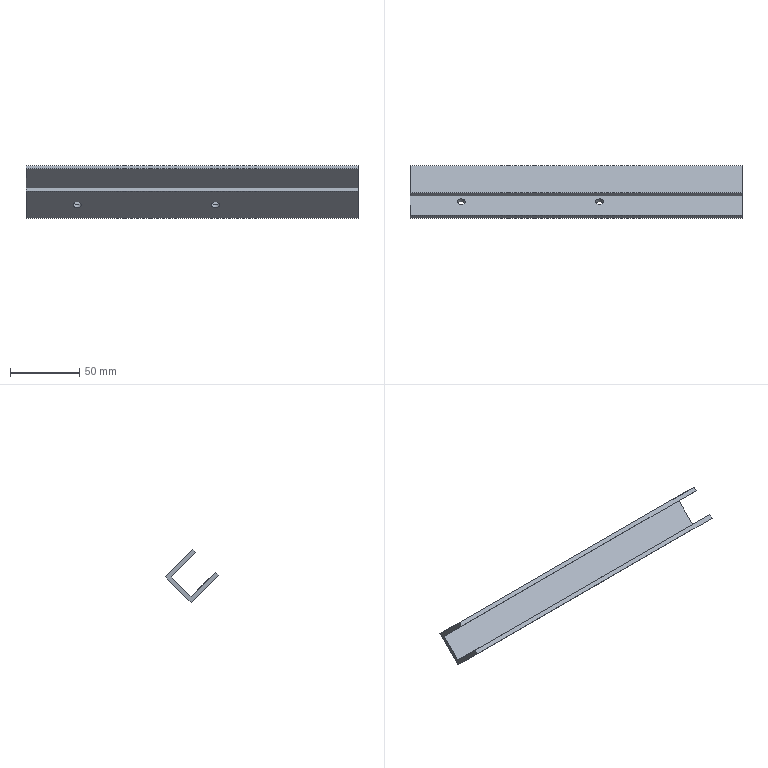Component | SolidWorks | Bracket-1 | 1 solid | 14 faces | box 240 x 38.18 x 38.18 mm | volume 54550 mm3 | plane 10 | cylinder 4 | commonest cylinder face diameters 6 x4
build123d program:
from build123d import *

# Parameters (mm, degrees)
EXTRUDE_THIN1_DEPTH = 240
SKETCH3_R           = 3
CUT_EXTRUDE1_DEPTH  = 3


with BuildPart() as part:
    # Sketch1 → Extrude-Thin1 (new body)
    with BuildSketch(Plane.XY):
        Polygon((-53.556, 14.33), (-25.556, 14.33), (-25.556, -11.67), (-53.556, -11.67), (-53.556, -8.67), (-28.556, -8.67), (-28.556, 11.33), (-53.556, 11.33), align=None)
    extrude(amount=EXTRUDE_THIN1_DEPTH)

    # Sketch3 → Cut-Extrude1 (cut)
    with BuildSketch(Plane(origin=(0, 14.33, 0), x_dir=(1, 0, 0), z_dir=(0, 1, 0))):
        with Locations(Location((-39.556, -103, 0), (0, 0, 270))):
            Circle(SKETCH3_R)
        with Locations(Location((-39.556, -203, 0), (0, 0, 270))):
            Circle(SKETCH3_R)
    extrude(amount=-CUT_EXTRUDE1_DEPTH, mode=Mode.SUBTRACT)


solid = part.part

# Placed as in the assembly
solid = solid.moved(Location((728.45, -151.935, -266.823), (-135, -90, 0)))
STEP:
#1=COLOUR_RGB('',0.7922,0.8196,0.9333);
#2=FILL_AREA_STYLE_COLOUR('',#1);
#3=FILL_AREA_STYLE('',(#2));
#4=SURFACE_STYLE_FILL_AREA(#3);
#5=SURFACE_SIDE_STYLE('',(#4));
#6=SURFACE_STYLE_USAGE(.BOTH.,#5);
#7=PRESENTATION_STYLE_ASSIGNMENT((#6));
#8=CARTESIAN_POINT('',(20.805,-7.398,-9.719));
#9=VERTEX_POINT('',#8);
#10=CARTESIAN_POINT('',(20.569,-7.398,-9.719));
#11=VERTEX_POINT('',#10);
#12=CARTESIAN_POINT('',(20.687,-7.398,-9.719));
#13=DIRECTION('',(0.,-0.7071,-0.7071));
#14=DIRECTION('',(-1.,0.,0.));
#15=AXIS2_PLACEMENT_3D('',#12,#13,#14);
#16=CIRCLE('',#15,0.1181);
#17=EDGE_CURVE('',#9,#11,#16,.T.);
#18=ORIENTED_EDGE('',*,*,#17,.F.);
#19=CARTESIAN_POINT('',(20.805,-7.482,-9.803));
#20=VERTEX_POINT('',#19);
#21=CARTESIAN_POINT('',(20.805,-7.398,-9.719));
#22=DIRECTION('',(0.,-0.7071,-0.7071));
#23=VECTOR('',#22,39.37);
#24=LINE('',#21,#23);
#25=EDGE_CURVE('',#9,#20,#24,.T.);
#26=ORIENTED_EDGE('',*,*,#25,.T.);
#27=CARTESIAN_POINT('',(20.569,-7.482,-9.803));
#28=VERTEX_POINT('',#27);
#29=CARTESIAN_POINT('',(20.687,-7.482,-9.803));
#30=DIRECTION('',(0.,-0.7071,-0.7071));
#31=DIRECTION('',(-1.,0.,0.));
#32=AXIS2_PLACEMENT_3D('',#29,#30,#31);
#33=CIRCLE('',#32,0.1181);
#34=EDGE_CURVE('',#20,#28,#33,.T.);
#35=ORIENTED_EDGE('',*,*,#34,.T.);
#36=CARTESIAN_POINT('',(20.569,-7.398,-9.719));
#37=DIRECTION('',(0.,-0.7071,-0.7071));
#38=VECTOR('',#37,39.37);
#39=LINE('',#36,#38);
#40=EDGE_CURVE('',#11,#28,#39,.T.);
#41=ORIENTED_EDGE('',*,*,#40,.F.);
#42=EDGE_LOOP('',(#18,#26,#35,#41));
#43=FACE_OUTER_BOUND('',#42,.T.);
#44=CARTESIAN_POINT('',(20.687,-7.398,-9.719));
#45=DIRECTION('',(0.,-0.7071,-0.7071));
#46=DIRECTION('',(-1.,0.,0.));
#47=AXIS2_PLACEMENT_3D('',#44,#45,#46);
#48=CYLINDRICAL_SURFACE('',#47,0.1181);
#49=ADVANCED_FACE('',(#43),#48,.F.);
#50=CARTESIAN_POINT('',(24.742,-7.398,-9.719));
#51=VERTEX_POINT('',#50);
#52=CARTESIAN_POINT('',(24.506,-7.398,-9.719));
#53=VERTEX_POINT('',#52);
#54=CARTESIAN_POINT('',(24.624,-7.398,-9.719));
#55=DIRECTION('',(0.,-0.7071,-0.7071));
#56=DIRECTION('',(-1.,0.,0.));
#57=AXIS2_PLACEMENT_3D('',#54,#55,#56);
#58=CIRCLE('',#57,0.1181);
#59=EDGE_CURVE('',#51,#53,#58,.T.);
#60=ORIENTED_EDGE('',*,*,#59,.F.);
#61=CARTESIAN_POINT('',(24.742,-7.482,-9.803));
#62=VERTEX_POINT('',#61);
#63=CARTESIAN_POINT('',(24.742,-7.398,-9.719));
#64=DIRECTION('',(0.,-0.7071,-0.7071));
#65=VECTOR('',#64,39.37);
#66=LINE('',#63,#65);
#67=EDGE_CURVE('',#51,#62,#66,.T.);
#68=ORIENTED_EDGE('',*,*,#67,.T.);
#69=CARTESIAN_POINT('',(24.506,-7.482,-9.803));
#70=VERTEX_POINT('',#69);
#71=CARTESIAN_POINT('',(24.624,-7.482,-9.803));
#72=DIRECTION('',(0.,-0.7071,-0.7071));
#73=DIRECTION('',(-1.,0.,0.));
#74=AXIS2_PLACEMENT_3D('',#71,#72,#73);
#75=CIRCLE('',#74,0.1181);
#76=EDGE_CURVE('',#62,#70,#75,.T.);
#77=ORIENTED_EDGE('',*,*,#76,.T.);
#78=CARTESIAN_POINT('',(24.506,-7.398,-9.719));
#79=DIRECTION('',(0.,-0.7071,-0.7071));
#80=VECTOR('',#79,39.37);
#81=LINE('',#78,#80);
#82=EDGE_CURVE('',#53,#70,#81,.T.);
#83=ORIENTED_EDGE('',*,*,#82,.F.);
#84=EDGE_LOOP('',(#60,#68,#77,#83));
#85=FACE_OUTER_BOUND('',#84,.T.);
#86=CARTESIAN_POINT('',(24.624,-7.398,-9.719));
#87=DIRECTION('',(0.,-0.7071,-0.7071));
#88=DIRECTION('',(-1.,0.,0.));
#89=AXIS2_PLACEMENT_3D('',#86,#87,#88);
#90=CYLINDRICAL_SURFACE('',#89,0.1181);
#91=ADVANCED_FACE('',(#85),#90,.F.);
#92=CARTESIAN_POINT('',(28.679,-6.535,-9.469));
#93=VERTEX_POINT('',#92);
#94=CARTESIAN_POINT('',(28.679,-7.231,-8.773));
#95=VERTEX_POINT('',#94);
#96=CARTESIAN_POINT('',(28.679,-6.452,-9.552));
#97=DIRECTION('',(-0.,-0.7071,0.7071));
#98=VECTOR('',#97,39.37);
#99=LINE('',#96,#98);
#100=EDGE_CURVE('',#93,#95,#99,.T.);
#101=ORIENTED_EDGE('',*,*,#100,.T.);
#102=CARTESIAN_POINT('',(19.23,-7.231,-8.773));
#103=VERTEX_POINT('',#102);
#104=CARTESIAN_POINT('',(19.23,-7.231,-8.773));
#105=DIRECTION('',(1.,-0.,0.));
#106=VECTOR('',#105,39.37);
#107=LINE('',#104,#106);
#108=EDGE_CURVE('',#103,#95,#107,.T.);
#109=ORIENTED_EDGE('',*,*,#108,.F.);
#110=CARTESIAN_POINT('',(19.23,-6.535,-9.469));
#111=VERTEX_POINT('',#110);
#112=CARTESIAN_POINT('',(19.23,-6.452,-9.552));
#113=DIRECTION('',(-0.,-0.7071,0.7071));
#114=VECTOR('',#113,39.37);
#115=LINE('',#112,#114);
#116=EDGE_CURVE('',#111,#103,#115,.T.);
#117=ORIENTED_EDGE('',*,*,#116,.F.);
#118=CARTESIAN_POINT('',(19.23,-6.535,-9.469));
#119=DIRECTION('',(1.,-0.,0.));
#120=VECTOR('',#119,39.37);
#121=LINE('',#118,#120);
#122=EDGE_CURVE('',#111,#93,#121,.T.);
#123=ORIENTED_EDGE('',*,*,#122,.T.);
#124=EDGE_LOOP('',(#101,#109,#117,#123));
#125=FACE_OUTER_BOUND('',#124,.T.);
#126=CARTESIAN_POINT('',(19.23,-6.452,-9.552));
#127=DIRECTION('',(-0.,0.7071,0.7071));
#128=DIRECTION('',(0.,0.7071,-0.7071));
#129=AXIS2_PLACEMENT_3D('',#126,#127,#128);
#130=PLANE('',#129);
#131=ADVANCED_FACE('',(#125),#130,.F.);
#132=CARTESIAN_POINT('',(28.679,-7.148,-8.689));
#133=VERTEX_POINT('',#132);
#134=CARTESIAN_POINT('',(28.679,-7.148,-8.689));
#135=DIRECTION('',(0.,-0.7071,-0.7071));
#136=VECTOR('',#135,39.37);
#137=LINE('',#134,#136);
#138=EDGE_CURVE('',#133,#95,#137,.T.);
#139=ORIENTED_EDGE('',*,*,#138,.F.);
#140=CARTESIAN_POINT('',(19.23,-7.148,-8.689));
#141=VERTEX_POINT('',#140);
#142=CARTESIAN_POINT('',(19.23,-7.148,-8.689));
#143=DIRECTION('',(1.,-0.,0.));
#144=VECTOR('',#143,39.37);
#145=LINE('',#142,#144);
#146=EDGE_CURVE('',#141,#133,#145,.T.);
#147=ORIENTED_EDGE('',*,*,#146,.F.);
#148=CARTESIAN_POINT('',(19.23,-7.148,-8.689));
#149=DIRECTION('',(0.,-0.7071,-0.7071));
#150=VECTOR('',#149,39.37);
#151=LINE('',#148,#150);
#152=EDGE_CURVE('',#141,#103,#151,.T.);
#153=ORIENTED_EDGE('',*,*,#152,.T.);
#154=ORIENTED_EDGE('',*,*,#108,.T.);
#155=EDGE_LOOP('',(#139,#147,#153,#154));
#156=FACE_OUTER_BOUND('',#155,.T.);
#157=CARTESIAN_POINT('',(19.23,-7.148,-8.689));
#158=DIRECTION('',(-0.,-0.7071,0.7071));
#159=DIRECTION('',(-1.,0.,-0.));
#160=AXIS2_PLACEMENT_3D('',#157,#158,#159);
#161=PLANE('',#160);
#162=ADVANCED_FACE('',(#156),#161,.T.);
#163=CARTESIAN_POINT('',(28.679,-6.368,-9.469));
#164=VERTEX_POINT('',#163);
#165=CARTESIAN_POINT('',(28.679,-6.368,-9.469));
#166=DIRECTION('',(-0.,-0.7071,0.7071));
#167=VECTOR('',#166,39.37);
#168=LINE('',#165,#167);
#169=EDGE_CURVE('',#164,#133,#168,.T.);
#170=ORIENTED_EDGE('',*,*,#169,.F.);
#171=CARTESIAN_POINT('',(19.23,-6.368,-9.469));
#172=VERTEX_POINT('',#171);
#173=CARTESIAN_POINT('',(19.23,-6.368,-9.469));
#174=DIRECTION('',(1.,-0.,0.));
#175=VECTOR('',#174,39.37);
#176=LINE('',#173,#175);
#177=EDGE_CURVE('',#172,#164,#176,.T.);
#178=ORIENTED_EDGE('',*,*,#177,.F.);
#179=CARTESIAN_POINT('',(19.23,-6.368,-9.469));
#180=DIRECTION('',(-0.,-0.7071,0.7071));
#181=VECTOR('',#180,39.37);
#182=LINE('',#179,#181);
#183=EDGE_CURVE('',#172,#141,#182,.T.);
#184=ORIENTED_EDGE('',*,*,#183,.T.);
#185=ORIENTED_EDGE('',*,*,#146,.T.);
#186=EDGE_LOOP('',(#170,#178,#184,#185));
#187=FACE_OUTER_BOUND('',#186,.T.);
#188=CARTESIAN_POINT('',(19.23,-6.368,-9.469));
#189=DIRECTION('',(-0.,0.7071,0.7071));
#190=DIRECTION('',(0.,0.7071,-0.7071));
#191=AXIS2_PLACEMENT_3D('',#188,#189,#190);
#192=PLANE('',#191);
#193=ADVANCED_FACE('',(#187),#192,.T.);
#194=CARTESIAN_POINT('',(28.679,-7.092,-10.192));
#195=VERTEX_POINT('',#194);
#196=CARTESIAN_POINT('',(28.679,-7.092,-10.192));
#197=DIRECTION('',(-0.,0.7071,0.7071));
#198=VECTOR('',#197,39.37);
#199=LINE('',#196,#198);
#200=EDGE_CURVE('',#195,#164,#199,.T.);
#201=ORIENTED_EDGE('',*,*,#200,.F.);
#202=CARTESIAN_POINT('',(19.23,-7.092,-10.192));
#203=VERTEX_POINT('',#202);
#204=CARTESIAN_POINT('',(19.23,-7.092,-10.192));
#205=DIRECTION('',(1.,-0.,0.));
#206=VECTOR('',#205,39.37);
#207=LINE('',#204,#206);
#208=EDGE_CURVE('',#203,#195,#207,.T.);
#209=ORIENTED_EDGE('',*,*,#208,.F.);
#210=CARTESIAN_POINT('',(19.23,-7.092,-10.192));
#211=DIRECTION('',(-0.,0.7071,0.7071));
#212=VECTOR('',#211,39.37);
#213=LINE('',#210,#212);
#214=EDGE_CURVE('',#203,#172,#213,.T.);
#215=ORIENTED_EDGE('',*,*,#214,.T.);
#216=ORIENTED_EDGE('',*,*,#177,.T.);
#217=EDGE_LOOP('',(#201,#209,#215,#216));
#218=FACE_OUTER_BOUND('',#217,.T.);
#219=CARTESIAN_POINT('',(19.23,-7.092,-10.192));
#220=DIRECTION('',(0.,0.7071,-0.7071));
#221=DIRECTION('',(1.,-0.,0.));
#222=AXIS2_PLACEMENT_3D('',#219,#220,#221);
#223=PLANE('',#222);
#224=ADVANCED_FACE('',(#218),#223,.T.);
#225=CARTESIAN_POINT('',(20.687,-7.482,-9.803));
#226=DIRECTION('',(0.,-0.7071,-0.7071));
#227=DIRECTION('',(-1.,0.,0.));
#228=AXIS2_PLACEMENT_3D('',#225,#226,#227);
#229=CIRCLE('',#228,0.1181);
#230=EDGE_CURVE('',#28,#20,#229,.T.);
#231=ORIENTED_EDGE('',*,*,#230,.F.);
#232=ORIENTED_EDGE('',*,*,#34,.F.);
#233=EDGE_LOOP('',(#231,#232));
#234=FACE_BOUND('',#233,.T.);
#235=CARTESIAN_POINT('',(24.624,-7.482,-9.803));
#236=DIRECTION('',(0.,-0.7071,-0.7071));
#237=DIRECTION('',(-1.,0.,0.));
#238=AXIS2_PLACEMENT_3D('',#235,#236,#237);
#239=CIRCLE('',#238,0.1181);
#240=EDGE_CURVE('',#70,#62,#239,.T.);
#241=ORIENTED_EDGE('',*,*,#240,.F.);
#242=ORIENTED_EDGE('',*,*,#76,.F.);
#243=EDGE_LOOP('',(#241,#242));
#244=FACE_BOUND('',#243,.T.);
#245=CARTESIAN_POINT('',(28.679,-7.872,-9.413));
#246=VERTEX_POINT('',#245);
#247=CARTESIAN_POINT('',(28.679,-7.872,-9.413));
#248=DIRECTION('',(0.,0.7071,-0.7071));
#249=VECTOR('',#248,39.37);
#250=LINE('',#247,#249);
#251=EDGE_CURVE('',#246,#195,#250,.T.);
#252=ORIENTED_EDGE('',*,*,#251,.F.);
#253=CARTESIAN_POINT('',(19.23,-7.872,-9.413));
#254=VERTEX_POINT('',#253);
#255=CARTESIAN_POINT('',(19.23,-7.872,-9.413));
#256=DIRECTION('',(1.,-0.,0.));
#257=VECTOR('',#256,39.37);
#258=LINE('',#255,#257);
#259=EDGE_CURVE('',#254,#246,#258,.T.);
#260=ORIENTED_EDGE('',*,*,#259,.F.);
#261=CARTESIAN_POINT('',(19.23,-7.872,-9.413));
#262=DIRECTION('',(0.,0.7071,-0.7071));
#263=VECTOR('',#262,39.37);
#264=LINE('',#261,#263);
#265=EDGE_CURVE('',#254,#203,#264,.T.);
#266=ORIENTED_EDGE('',*,*,#265,.T.);
#267=ORIENTED_EDGE('',*,*,#208,.T.);
#268=EDGE_LOOP('',(#252,#260,#266,#267));
#269=FACE_OUTER_BOUND('',#268,.T.);
#270=CARTESIAN_POINT('',(19.23,-7.872,-9.413));
#271=DIRECTION('',(0.,-0.7071,-0.7071));
#272=DIRECTION('',(-1.,0.,-0.));
#273=AXIS2_PLACEMENT_3D('',#270,#271,#272);
#274=PLANE('',#273);
#275=ADVANCED_FACE('',(#234,#244,#269),#274,.T.);
#276=CARTESIAN_POINT('',(28.679,-7.788,-9.329));
#277=VERTEX_POINT('',#276);
#278=CARTESIAN_POINT('',(28.679,-7.788,-9.329));
#279=DIRECTION('',(0.,-0.7071,-0.7071));
#280=VECTOR('',#279,39.37);
#281=LINE('',#278,#280);
#282=EDGE_CURVE('',#277,#246,#281,.T.);
#283=ORIENTED_EDGE('',*,*,#282,.F.);
#284=CARTESIAN_POINT('',(19.23,-7.788,-9.329));
#285=VERTEX_POINT('',#284);
#286=CARTESIAN_POINT('',(19.23,-7.788,-9.329));
#287=DIRECTION('',(1.,-0.,0.));
#288=VECTOR('',#287,39.37);
#289=LINE('',#286,#288);
#290=EDGE_CURVE('',#285,#277,#289,.T.);
#291=ORIENTED_EDGE('',*,*,#290,.F.);
#292=CARTESIAN_POINT('',(19.23,-7.788,-9.329));
#293=DIRECTION('',(0.,-0.7071,-0.7071));
#294=VECTOR('',#293,39.37);
#295=LINE('',#292,#294);
#296=EDGE_CURVE('',#285,#254,#295,.T.);
#297=ORIENTED_EDGE('',*,*,#296,.T.);
#298=ORIENTED_EDGE('',*,*,#259,.T.);
#299=EDGE_LOOP('',(#283,#291,#297,#298));
#300=FACE_OUTER_BOUND('',#299,.T.);
#301=CARTESIAN_POINT('',(19.23,-7.788,-9.329));
#302=DIRECTION('',(-0.,-0.7071,0.7071));
#303=DIRECTION('',(-1.,0.,-0.));
#304=AXIS2_PLACEMENT_3D('',#301,#302,#303);
#305=PLANE('',#304);
#306=ADVANCED_FACE('',(#300),#305,.T.);
#307=CARTESIAN_POINT('',(20.687,-7.398,-9.719));
#308=DIRECTION('',(0.,-0.7071,-0.7071));
#309=DIRECTION('',(-1.,0.,0.));
#310=AXIS2_PLACEMENT_3D('',#307,#308,#309);
#311=CIRCLE('',#310,0.1181);
#312=EDGE_CURVE('',#11,#9,#311,.T.);
#313=ORIENTED_EDGE('',*,*,#312,.T.);
#314=ORIENTED_EDGE('',*,*,#17,.T.);
#315=EDGE_LOOP('',(#313,#314));
#316=FACE_BOUND('',#315,.T.);
#317=CARTESIAN_POINT('',(24.624,-7.398,-9.719));
#318=DIRECTION('',(0.,-0.7071,-0.7071));
#319=DIRECTION('',(-1.,0.,0.));
#320=AXIS2_PLACEMENT_3D('',#317,#318,#319);
#321=CIRCLE('',#320,0.1181);
#322=EDGE_CURVE('',#53,#51,#321,.T.);
#323=ORIENTED_EDGE('',*,*,#322,.T.);
#324=ORIENTED_EDGE('',*,*,#59,.T.);
#325=EDGE_LOOP('',(#323,#324));
#326=FACE_BOUND('',#325,.T.);
#327=CARTESIAN_POINT('',(28.679,-7.092,-10.025));
#328=VERTEX_POINT('',#327);
#329=CARTESIAN_POINT('',(28.679,-7.788,-9.329));
#330=DIRECTION('',(0.,0.7071,-0.7071));
#331=VECTOR('',#330,39.37);
#332=LINE('',#329,#331);
#333=EDGE_CURVE('',#277,#328,#332,.T.);
#334=ORIENTED_EDGE('',*,*,#333,.T.);
#335=CARTESIAN_POINT('',(19.23,-7.092,-10.025));
#336=VERTEX_POINT('',#335);
#337=CARTESIAN_POINT('',(19.23,-7.092,-10.025));
#338=DIRECTION('',(1.,-0.,0.));
#339=VECTOR('',#338,39.37);
#340=LINE('',#337,#339);
#341=EDGE_CURVE('',#336,#328,#340,.T.);
#342=ORIENTED_EDGE('',*,*,#341,.F.);
#343=CARTESIAN_POINT('',(19.23,-7.788,-9.329));
#344=DIRECTION('',(0.,0.7071,-0.7071));
#345=VECTOR('',#344,39.37);
#346=LINE('',#343,#345);
#347=EDGE_CURVE('',#285,#336,#346,.T.);
#348=ORIENTED_EDGE('',*,*,#347,.F.);
#349=ORIENTED_EDGE('',*,*,#290,.T.);
#350=EDGE_LOOP('',(#334,#342,#348,#349));
#351=FACE_OUTER_BOUND('',#350,.T.);
#352=CARTESIAN_POINT('',(19.23,-7.788,-9.329));
#353=DIRECTION('',(0.,-0.7071,-0.7071));
#354=DIRECTION('',(-1.,0.,-0.));
#355=AXIS2_PLACEMENT_3D('',#352,#353,#354);
#356=PLANE('',#355);
#357=ADVANCED_FACE('',(#316,#326,#351),#356,.F.);
#358=CARTESIAN_POINT('',(28.679,-7.176,-10.109));
#359=DIRECTION('',(-0.,0.7071,0.7071));
#360=VECTOR('',#359,39.37);
#361=LINE('',#358,#360);
#362=EDGE_CURVE('',#328,#93,#361,.T.);
#363=ORIENTED_EDGE('',*,*,#362,.T.);
#364=ORIENTED_EDGE('',*,*,#122,.F.);
#365=CARTESIAN_POINT('',(19.23,-7.176,-10.109));
#366=DIRECTION('',(-0.,0.7071,0.7071));
#367=VECTOR('',#366,39.37);
#368=LINE('',#365,#367);
#369=EDGE_CURVE('',#336,#111,#368,.T.);
#370=ORIENTED_EDGE('',*,*,#369,.F.);
#371=ORIENTED_EDGE('',*,*,#341,.T.);
#372=EDGE_LOOP('',(#363,#364,#370,#371));
#373=FACE_OUTER_BOUND('',#372,.T.);
#374=CARTESIAN_POINT('',(19.23,-7.176,-10.109));
#375=DIRECTION('',(0.,0.7071,-0.7071));
#376=DIRECTION('',(1.,-0.,0.));
#377=AXIS2_PLACEMENT_3D('',#374,#375,#376);
#378=PLANE('',#377);
#379=ADVANCED_FACE('',(#373),#378,.F.);
#380=ORIENTED_EDGE('',*,*,#116,.T.);
#381=ORIENTED_EDGE('',*,*,#152,.F.);
#382=ORIENTED_EDGE('',*,*,#183,.F.);
#383=ORIENTED_EDGE('',*,*,#214,.F.);
#384=ORIENTED_EDGE('',*,*,#265,.F.);
#385=ORIENTED_EDGE('',*,*,#296,.F.);
#386=ORIENTED_EDGE('',*,*,#347,.T.);
#387=ORIENTED_EDGE('',*,*,#369,.T.);
#388=EDGE_LOOP('',(#380,#381,#382,#383,#384,#385,#386,#387));
#389=FACE_OUTER_BOUND('',#388,.T.);
#390=CARTESIAN_POINT('',(19.23,-5.982,-10.505));
#391=DIRECTION('',(1.,-0.,0.));
#392=DIRECTION('',(-0.,-0.7071,0.7071));
#393=AXIS2_PLACEMENT_3D('',#390,#391,#392);
#394=PLANE('',#393);
#395=ADVANCED_FACE('',(#389),#394,.F.);
#396=ORIENTED_EDGE('',*,*,#100,.F.);
#397=ORIENTED_EDGE('',*,*,#362,.F.);
#398=ORIENTED_EDGE('',*,*,#333,.F.);
#399=ORIENTED_EDGE('',*,*,#282,.T.);
#400=ORIENTED_EDGE('',*,*,#251,.T.);
#401=ORIENTED_EDGE('',*,*,#200,.T.);
#402=ORIENTED_EDGE('',*,*,#169,.T.);
#403=ORIENTED_EDGE('',*,*,#138,.T.);
#404=EDGE_LOOP('',(#396,#397,#398,#399,#400,#401,#402,#403));
#405=FACE_OUTER_BOUND('',#404,.T.);
#406=CARTESIAN_POINT('',(28.679,-5.982,-10.505));
#407=DIRECTION('',(1.,-0.,0.));
#408=DIRECTION('',(-0.,-0.7071,0.7071));
#409=AXIS2_PLACEMENT_3D('',#406,#407,#408);
#410=PLANE('',#409);
#411=ADVANCED_FACE('',(#405),#410,.T.);
#412=ORIENTED_EDGE('',*,*,#67,.F.);
#413=ORIENTED_EDGE('',*,*,#322,.F.);
#414=ORIENTED_EDGE('',*,*,#82,.T.);
#415=ORIENTED_EDGE('',*,*,#240,.T.);
#416=EDGE_LOOP('',(#412,#413,#414,#415));
#417=FACE_OUTER_BOUND('',#416,.T.);
#418=CARTESIAN_POINT('',(24.624,-7.398,-9.719));
#419=DIRECTION('',(0.,-0.7071,-0.7071));
#420=DIRECTION('',(-1.,0.,0.));
#421=AXIS2_PLACEMENT_3D('',#418,#419,#420);
#422=CYLINDRICAL_SURFACE('',#421,0.1181);
#423=ADVANCED_FACE('',(#417),#422,.F.);
#424=ORIENTED_EDGE('',*,*,#25,.F.);
#425=ORIENTED_EDGE('',*,*,#312,.F.);
#426=ORIENTED_EDGE('',*,*,#40,.T.);
#427=ORIENTED_EDGE('',*,*,#230,.T.);
#428=EDGE_LOOP('',(#424,#425,#426,#427));
#429=FACE_OUTER_BOUND('',#428,.T.);
#430=CARTESIAN_POINT('',(20.687,-7.398,-9.719));
#431=DIRECTION('',(0.,-0.7071,-0.7071));
#432=DIRECTION('',(-1.,0.,0.));
#433=AXIS2_PLACEMENT_3D('',#430,#431,#432);
#434=CYLINDRICAL_SURFACE('',#433,0.1181);
#435=ADVANCED_FACE('',(#429),#434,.F.);
#436=CLOSED_SHELL('',(#49,#91,#131,#162,#193,#224,#275,#306,#357,#379,#395,#411,#423,#435));
#437=MANIFOLD_SOLID_BREP('',#436);
#438=STYLED_ITEM('',(#7),#437);
#439=PRESENTATION_LAYER_ASSIGNMENT('','',(#438));
#440=(LENGTH_UNIT()NAMED_UNIT(*)SI_UNIT($,.METRE.));
#441=LENGTH_MEASURE_WITH_UNIT(LENGTH_MEASURE(0.0254),#440);
#442=DIMENSIONAL_EXPONENTS(1.,0.,0.,0.,0.,0.,0.);
#443=(CONVERSION_BASED_UNIT('',#441)LENGTH_UNIT()NAMED_UNIT(#442));
#444=UNCERTAINTY_MEASURE_WITH_UNIT(LENGTH_MEASURE(0.00001),#443,'','');
#445=(NAMED_UNIT(*)PLANE_ANGLE_UNIT()SI_UNIT($,.RADIAN.));
#446=(NAMED_UNIT(*)SI_UNIT($,.STERADIAN.)SOLID_ANGLE_UNIT());
#447=(GEOMETRIC_REPRESENTATION_CONTEXT(3)GLOBAL_UNCERTAINTY_ASSIGNED_CONTEXT((#444))GLOBAL_UNIT_ASSIGNED_CONTEXT((#443,#445,#446))REPRESENTATION_CONTEXT('',''));
#448=MECHANICAL_DESIGN_GEOMETRIC_PRESENTATION_REPRESENTATION('',(#438),#447);
#449=CARTESIAN_POINT('',(0.,0.,0.));
#450=DIRECTION('',(0.,0.,1.));
#451=DIRECTION('',(1.,0.,0.));
#452=AXIS2_PLACEMENT_3D('',#449,#450,#451);
#453=(LENGTH_UNIT()NAMED_UNIT(*)SI_UNIT($,.METRE.));
#454=LENGTH_MEASURE_WITH_UNIT(LENGTH_MEASURE(0.0254),#453);
#455=DIMENSIONAL_EXPONENTS(1.,0.,0.,0.,0.,0.,0.);
#456=(CONVERSION_BASED_UNIT('',#454)LENGTH_UNIT()NAMED_UNIT(#455));
#457=UNCERTAINTY_MEASURE_WITH_UNIT(LENGTH_MEASURE(0.00001),#456,'','');
#458=(NAMED_UNIT(*)PLANE_ANGLE_UNIT()SI_UNIT($,.RADIAN.));
#459=(NAMED_UNIT(*)SI_UNIT($,.STERADIAN.)SOLID_ANGLE_UNIT());
#460=(GEOMETRIC_REPRESENTATION_CONTEXT(3)GLOBAL_UNCERTAINTY_ASSIGNED_CONTEXT((#457))GLOBAL_UNIT_ASSIGNED_CONTEXT((#456,#458,#459))REPRESENTATION_CONTEXT('',''));
#461=ADVANCED_BREP_SHAPE_REPRESENTATION('',(#437,#452),#460);